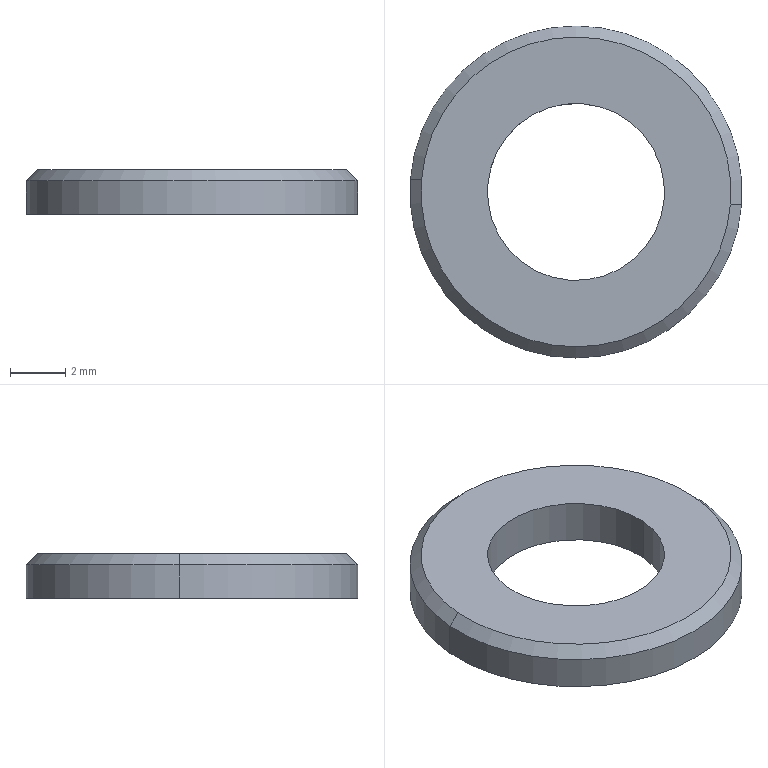Component | SolidWorks | WasherM6-1 | 1 solid | 8 faces | box 12 x 12 x 1.6 mm | volume 127 mm3 | cylinder 4 | cone 2 | plane 2 | commonest cylinder face diameters 6.4 x2 12 x2
build123d program:
from build123d import *

# Parameters (mm, degrees)
SKETCH1_R          = 6
SKETCH1_R_2        = 3.2
BASE_EXTRUDE_DEPTH = 1.6
CHAMFER1_SIZE      = 0.4


with BuildPart() as part:
    # Sketch1 → Base-Extrude (new body)
    with BuildSketch(Plane.XY):
        Circle(SKETCH1_R)
        Circle(SKETCH1_R_2, mode=Mode.SUBTRACT)
    extrude(amount=-BASE_EXTRUDE_DEPTH)

    # Chamfer1
    chamfer1_edges = [part.edges().sort_by_distance(p)[0] for p in [
        (-6, 0, 0),
    ]]
    chamfer(chamfer1_edges, length=CHAMFER1_SIZE)


solid = part.part

# Placed as in the assembly
solid = solid.moved(Location((-15.928, -1.7, 16.655), (0, 0, 0)))
STEP:
#1=COLOUR_RGB('',0.7922,0.8196,0.9333);
#2=FILL_AREA_STYLE_COLOUR('',#1);
#3=FILL_AREA_STYLE('',(#2));
#4=SURFACE_STYLE_FILL_AREA(#3);
#5=SURFACE_SIDE_STYLE('',(#4));
#6=SURFACE_STYLE_USAGE(.BOTH.,#5);
#7=PRESENTATION_STYLE_ASSIGNMENT((#6));
#8=CARTESIAN_POINT('',(-0.4073,-0.08405,0.6557));
#9=VERTEX_POINT('',#8);
#10=CARTESIAN_POINT('',(-0.8469,-0.04982,0.6557));
#11=VERTEX_POINT('',#10);
#12=CARTESIAN_POINT('',(-0.6271,-0.06694,0.6557));
#13=DIRECTION('',(0.,0.,1.));
#14=DIRECTION('',(0.997,-0.07762,0.));
#15=AXIS2_PLACEMENT_3D('',#12,#13,#14);
#16=CIRCLE('',#15,0.2205);
#17=EDGE_CURVE('',#9,#11,#16,.T.);
#18=ORIENTED_EDGE('',*,*,#17,.F.);
#19=CARTESIAN_POINT('',(-0.3916,-0.08527,0.64));
#20=VERTEX_POINT('',#19);
#21=CARTESIAN_POINT('',(-0.4073,-0.08405,0.6557));
#22=DIRECTION('',(0.705,-0.05488,-0.7071));
#23=VECTOR('',#22,39.37);
#24=LINE('',#21,#23);
#25=EDGE_CURVE('',#9,#20,#24,.T.);
#26=ORIENTED_EDGE('',*,*,#25,.T.);
#27=CARTESIAN_POINT('',(-0.8626,-0.0486,0.64));
#28=VERTEX_POINT('',#27);
#29=CARTESIAN_POINT('',(-0.6271,-0.06694,0.64));
#30=DIRECTION('',(0.,0.,-1.));
#31=DIRECTION('',(0.997,-0.07762,0.));
#32=AXIS2_PLACEMENT_3D('',#29,#30,#31);
#33=CIRCLE('',#32,0.2362);
#34=EDGE_CURVE('',#28,#20,#33,.T.);
#35=ORIENTED_EDGE('',*,*,#34,.F.);
#36=CARTESIAN_POINT('',(-0.8469,-0.04982,0.6557));
#37=DIRECTION('',(-0.705,0.05488,-0.7071));
#38=VECTOR('',#37,39.37);
#39=LINE('',#36,#38);
#40=EDGE_CURVE('',#11,#28,#39,.T.);
#41=ORIENTED_EDGE('',*,*,#40,.F.);
#42=EDGE_LOOP('',(#18,#26,#35,#41));
#43=FACE_OUTER_BOUND('',#42,.T.);
#44=CARTESIAN_POINT('',(-0.6271,-0.06694,0.6557));
#45=DIRECTION('',(0.,0.,-1.));
#46=DIRECTION('',(-0.997,0.07762,0.));
#47=AXIS2_PLACEMENT_3D('',#44,#45,#46);
#48=CONICAL_SURFACE('',#47,0.2205,0.7854);
#49=ADVANCED_FACE('',(#43),#48,.T.);
#50=CARTESIAN_POINT('',(-0.7527,-0.05716,0.5927));
#51=VERTEX_POINT('',#50);
#52=CARTESIAN_POINT('',(-0.5015,-0.07672,0.5927));
#53=VERTEX_POINT('',#52);
#54=CARTESIAN_POINT('',(-0.6271,-0.06694,0.5927));
#55=DIRECTION('',(0.,0.,1.));
#56=DIRECTION('',(0.997,-0.07762,0.));
#57=AXIS2_PLACEMENT_3D('',#54,#55,#56);
#58=CIRCLE('',#57,0.126);
#59=EDGE_CURVE('',#51,#53,#58,.T.);
#60=ORIENTED_EDGE('',*,*,#59,.F.);
#61=CARTESIAN_POINT('',(-0.7527,-0.05716,0.6557));
#62=VERTEX_POINT('',#61);
#63=CARTESIAN_POINT('',(-0.7527,-0.05716,0.5927));
#64=DIRECTION('',(0.,0.,1.));
#65=VECTOR('',#64,39.37);
#66=LINE('',#63,#65);
#67=EDGE_CURVE('',#51,#62,#66,.T.);
#68=ORIENTED_EDGE('',*,*,#67,.T.);
#69=CARTESIAN_POINT('',(-0.5015,-0.07672,0.6557));
#70=VERTEX_POINT('',#69);
#71=CARTESIAN_POINT('',(-0.6271,-0.06694,0.6557));
#72=DIRECTION('',(0.,0.,1.));
#73=DIRECTION('',(0.997,-0.07762,0.));
#74=AXIS2_PLACEMENT_3D('',#71,#72,#73);
#75=CIRCLE('',#74,0.126);
#76=EDGE_CURVE('',#62,#70,#75,.T.);
#77=ORIENTED_EDGE('',*,*,#76,.T.);
#78=CARTESIAN_POINT('',(-0.5015,-0.07672,0.5927));
#79=DIRECTION('',(0.,0.,1.));
#80=VECTOR('',#79,39.37);
#81=LINE('',#78,#80);
#82=EDGE_CURVE('',#53,#70,#81,.T.);
#83=ORIENTED_EDGE('',*,*,#82,.F.);
#84=EDGE_LOOP('',(#60,#68,#77,#83));
#85=FACE_OUTER_BOUND('',#84,.T.);
#86=CARTESIAN_POINT('',(-0.6271,-0.06694,0.5927));
#87=DIRECTION('',(0.,0.,1.));
#88=DIRECTION('',(0.997,-0.07762,0.));
#89=AXIS2_PLACEMENT_3D('',#86,#87,#88);
#90=CYLINDRICAL_SURFACE('',#89,0.126);
#91=ADVANCED_FACE('',(#85),#90,.F.);
#92=CARTESIAN_POINT('',(-0.3916,-0.08527,0.5927));
#93=VERTEX_POINT('',#92);
#94=CARTESIAN_POINT('',(-0.8626,-0.0486,0.5927));
#95=VERTEX_POINT('',#94);
#96=CARTESIAN_POINT('',(-0.6271,-0.06694,0.5927));
#97=DIRECTION('',(0.,0.,1.));
#98=DIRECTION('',(0.997,-0.07762,0.));
#99=AXIS2_PLACEMENT_3D('',#96,#97,#98);
#100=CIRCLE('',#99,0.2362);
#101=EDGE_CURVE('',#93,#95,#100,.T.);
#102=ORIENTED_EDGE('',*,*,#101,.T.);
#103=CARTESIAN_POINT('',(-0.8626,-0.0486,0.5927));
#104=DIRECTION('',(0.,0.,1.));
#105=VECTOR('',#104,39.37);
#106=LINE('',#103,#105);
#107=EDGE_CURVE('',#95,#28,#106,.T.);
#108=ORIENTED_EDGE('',*,*,#107,.T.);
#109=ORIENTED_EDGE('',*,*,#34,.T.);
#110=CARTESIAN_POINT('',(-0.3916,-0.08527,0.5927));
#111=DIRECTION('',(0.,0.,1.));
#112=VECTOR('',#111,39.37);
#113=LINE('',#110,#112);
#114=EDGE_CURVE('',#93,#20,#113,.T.);
#115=ORIENTED_EDGE('',*,*,#114,.F.);
#116=EDGE_LOOP('',(#102,#108,#109,#115));
#117=FACE_OUTER_BOUND('',#116,.T.);
#118=CARTESIAN_POINT('',(-0.6271,-0.06694,0.5927));
#119=DIRECTION('',(0.,0.,1.));
#120=DIRECTION('',(0.997,-0.07762,0.));
#121=AXIS2_PLACEMENT_3D('',#118,#119,#120);
#122=CYLINDRICAL_SURFACE('',#121,0.2362);
#123=ADVANCED_FACE('',(#117),#122,.T.);
#124=ORIENTED_EDGE('',*,*,#107,.F.);
#125=CARTESIAN_POINT('',(-0.6271,-0.06694,0.5927));
#126=DIRECTION('',(0.,0.,1.));
#127=DIRECTION('',(0.997,-0.07762,0.));
#128=AXIS2_PLACEMENT_3D('',#125,#126,#127);
#129=CIRCLE('',#128,0.2362);
#130=EDGE_CURVE('',#95,#93,#129,.T.);
#131=ORIENTED_EDGE('',*,*,#130,.T.);
#132=ORIENTED_EDGE('',*,*,#114,.T.);
#133=CARTESIAN_POINT('',(-0.6271,-0.06694,0.64));
#134=DIRECTION('',(0.,0.,-1.));
#135=DIRECTION('',(0.997,-0.07762,0.));
#136=AXIS2_PLACEMENT_3D('',#133,#134,#135);
#137=CIRCLE('',#136,0.2362);
#138=EDGE_CURVE('',#20,#28,#137,.T.);
#139=ORIENTED_EDGE('',*,*,#138,.T.);
#140=EDGE_LOOP('',(#124,#131,#132,#139));
#141=FACE_OUTER_BOUND('',#140,.T.);
#142=CARTESIAN_POINT('',(-0.6271,-0.06694,0.5927));
#143=DIRECTION('',(0.,0.,1.));
#144=DIRECTION('',(0.997,-0.07762,0.));
#145=AXIS2_PLACEMENT_3D('',#142,#143,#144);
#146=CYLINDRICAL_SURFACE('',#145,0.2362);
#147=ADVANCED_FACE('',(#141),#146,.T.);
#148=CARTESIAN_POINT('',(-0.6271,-0.06694,0.5927));
#149=DIRECTION('',(0.,0.,1.));
#150=DIRECTION('',(0.997,-0.07762,0.));
#151=AXIS2_PLACEMENT_3D('',#148,#149,#150);
#152=CIRCLE('',#151,0.126);
#153=EDGE_CURVE('',#53,#51,#152,.T.);
#154=ORIENTED_EDGE('',*,*,#153,.T.);
#155=ORIENTED_EDGE('',*,*,#59,.T.);
#156=EDGE_LOOP('',(#154,#155));
#157=FACE_BOUND('',#156,.T.);
#158=ORIENTED_EDGE('',*,*,#101,.F.);
#159=ORIENTED_EDGE('',*,*,#130,.F.);
#160=EDGE_LOOP('',(#158,#159));
#161=FACE_OUTER_BOUND('',#160,.T.);
#162=CARTESIAN_POINT('',(-0.6271,-0.06694,0.5927));
#163=DIRECTION('',(0.,0.,1.));
#164=DIRECTION('',(0.997,-0.07762,0.));
#165=AXIS2_PLACEMENT_3D('',#162,#163,#164);
#166=PLANE('',#165);
#167=ADVANCED_FACE('',(#157,#161),#166,.F.);
#168=CARTESIAN_POINT('',(-0.6271,-0.06694,0.6557));
#169=DIRECTION('',(0.,0.,1.));
#170=DIRECTION('',(0.997,-0.07762,0.));
#171=AXIS2_PLACEMENT_3D('',#168,#169,#170);
#172=CIRCLE('',#171,0.2205);
#173=EDGE_CURVE('',#11,#9,#172,.T.);
#174=ORIENTED_EDGE('',*,*,#173,.T.);
#175=ORIENTED_EDGE('',*,*,#17,.T.);
#176=EDGE_LOOP('',(#174,#175));
#177=FACE_OUTER_BOUND('',#176,.T.);
#178=CARTESIAN_POINT('',(-0.6271,-0.06694,0.6557));
#179=DIRECTION('',(0.,0.,1.));
#180=DIRECTION('',(0.997,-0.07762,0.));
#181=AXIS2_PLACEMENT_3D('',#178,#179,#180);
#182=CIRCLE('',#181,0.126);
#183=EDGE_CURVE('',#70,#62,#182,.T.);
#184=ORIENTED_EDGE('',*,*,#183,.F.);
#185=ORIENTED_EDGE('',*,*,#76,.F.);
#186=EDGE_LOOP('',(#184,#185));
#187=FACE_BOUND('',#186,.T.);
#188=CARTESIAN_POINT('',(-0.6271,-0.06694,0.6557));
#189=DIRECTION('',(0.,0.,1.));
#190=DIRECTION('',(0.997,-0.07762,0.));
#191=AXIS2_PLACEMENT_3D('',#188,#189,#190);
#192=PLANE('',#191);
#193=ADVANCED_FACE('',(#177,#187),#192,.T.);
#194=ORIENTED_EDGE('',*,*,#67,.F.);
#195=ORIENTED_EDGE('',*,*,#153,.F.);
#196=ORIENTED_EDGE('',*,*,#82,.T.);
#197=ORIENTED_EDGE('',*,*,#183,.T.);
#198=EDGE_LOOP('',(#194,#195,#196,#197));
#199=FACE_OUTER_BOUND('',#198,.T.);
#200=CARTESIAN_POINT('',(-0.6271,-0.06694,0.5927));
#201=DIRECTION('',(0.,0.,1.));
#202=DIRECTION('',(0.997,-0.07762,0.));
#203=AXIS2_PLACEMENT_3D('',#200,#201,#202);
#204=CYLINDRICAL_SURFACE('',#203,0.126);
#205=ADVANCED_FACE('',(#199),#204,.F.);
#206=ORIENTED_EDGE('',*,*,#25,.F.);
#207=ORIENTED_EDGE('',*,*,#173,.F.);
#208=ORIENTED_EDGE('',*,*,#40,.T.);
#209=ORIENTED_EDGE('',*,*,#138,.F.);
#210=EDGE_LOOP('',(#206,#207,#208,#209));
#211=FACE_OUTER_BOUND('',#210,.T.);
#212=CARTESIAN_POINT('',(-0.6271,-0.06694,0.6557));
#213=DIRECTION('',(0.,0.,-1.));
#214=DIRECTION('',(-0.997,0.07762,0.));
#215=AXIS2_PLACEMENT_3D('',#212,#213,#214);
#216=CONICAL_SURFACE('',#215,0.2205,0.7854);
#217=ADVANCED_FACE('',(#211),#216,.T.);
#218=CLOSED_SHELL('',(#49,#91,#123,#147,#167,#193,#205,#217));
#219=MANIFOLD_SOLID_BREP('',#218);
#220=STYLED_ITEM('',(#7),#219);
#221=PRESENTATION_LAYER_ASSIGNMENT('','',(#220));
#222=CARTESIAN_POINT('',(0.,0.,0.));
#223=DIRECTION('',(0.,0.,1.));
#224=DIRECTION('',(1.,0.,0.));
#225=AXIS2_PLACEMENT_3D('',#222,#223,#224);
#226=(LENGTH_UNIT()NAMED_UNIT(*)SI_UNIT($,.METRE.));
#227=LENGTH_MEASURE_WITH_UNIT(LENGTH_MEASURE(0.0254),#226);
#228=DIMENSIONAL_EXPONENTS(1.,0.,0.,0.,0.,0.,0.);
#229=(CONVERSION_BASED_UNIT('',#227)LENGTH_UNIT()NAMED_UNIT(#228));
#230=UNCERTAINTY_MEASURE_WITH_UNIT(LENGTH_MEASURE(0.00001),#229,'','');
#231=(NAMED_UNIT(*)PLANE_ANGLE_UNIT()SI_UNIT($,.RADIAN.));
#232=(NAMED_UNIT(*)SI_UNIT($,.STERADIAN.)SOLID_ANGLE_UNIT());
#233=(GEOMETRIC_REPRESENTATION_CONTEXT(3)GLOBAL_UNCERTAINTY_ASSIGNED_CONTEXT((#230))GLOBAL_UNIT_ASSIGNED_CONTEXT((#229,#231,#232))REPRESENTATION_CONTEXT('',''));
#234=ADVANCED_BREP_SHAPE_REPRESENTATION('',(#219,#225),#233);
#235=(LENGTH_UNIT()NAMED_UNIT(*)SI_UNIT($,.METRE.));
#236=LENGTH_MEASURE_WITH_UNIT(LENGTH_MEASURE(0.0254),#235);
#237=DIMENSIONAL_EXPONENTS(1.,0.,0.,0.,0.,0.,0.);
#238=(CONVERSION_BASED_UNIT('',#236)LENGTH_UNIT()NAMED_UNIT(#237));
#239=UNCERTAINTY_MEASURE_WITH_UNIT(LENGTH_MEASURE(0.00001),#238,'','');
#240=(NAMED_UNIT(*)PLANE_ANGLE_UNIT()SI_UNIT($,.RADIAN.));
#241=(NAMED_UNIT(*)SI_UNIT($,.STERADIAN.)SOLID_ANGLE_UNIT());
#242=(GEOMETRIC_REPRESENTATION_CONTEXT(3)GLOBAL_UNCERTAINTY_ASSIGNED_CONTEXT((#239))GLOBAL_UNIT_ASSIGNED_CONTEXT((#238,#240,#241))REPRESENTATION_CONTEXT('',''));
#243=MECHANICAL_DESIGN_GEOMETRIC_PRESENTATION_REPRESENTATION('',(#220),#242);